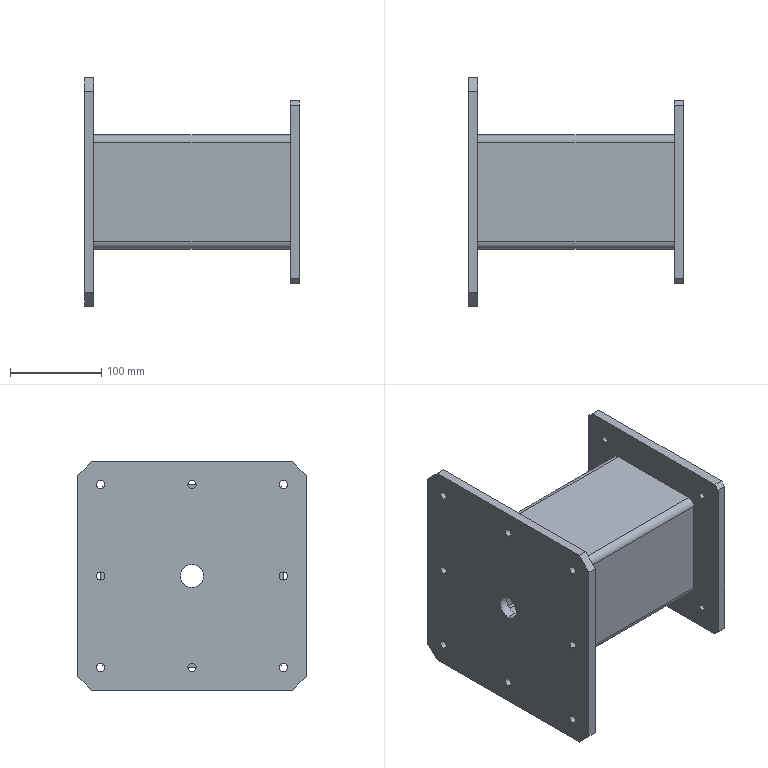Component | SolidWorks | Base-1 | 1 solid | 66 faces | box 235 x 250 x 250 mm | volume 1606520 mm3 | cylinder 36 | plane 30 | commonest cylinder face diameters 9 x16 7 x8 25 x4 16 x4 4 x4 | material Plain Carbon Steel
build123d program:
from build123d import *

# Parameters (mm, degrees)
SKETCH1_W                 = 400
SKETCH1_H                 = 400
BOSS_EXTRUDE1_DEPTH       = 20
BOSS_EXTRUDE2_DEPTH       = 430
SKETCH3_W                 = 500
SKETCH3_H                 = 500
BOSS_EXTRUDE3_DEPTH       = 20
CHAMFER1_SIZE             = 30
CHAMFER2_SIZE             = 10
M16_TAPPED_HOLE1_REACH    = 590.133
M16_TAPPED_HOLE1_BORE_R   = 7
M16_CLEARANCE_HOLE1_D     = 18
M16_CLEARANCE_HOLE1_DEPTH = 20
CUT_EXTRUDE1_DEPTH        = 589.133
CUT_EXTRUDE1_DEPTH_BACK   = 589.133
SKETCH11_R                = 25
SCALE1_SCALE              = 0.5


with BuildPart() as part:
    # Sketch1 → Boss-Extrude1 (new body)
    with BuildSketch(Plane.XY):
        Rectangle(SKETCH1_W, SKETCH1_H)
    extrude(amount=BOSS_EXTRUDE1_DEPTH)

    # Sketch2 → Boss-Extrude2 (add)
    with BuildSketch(Plane(origin=(0, 0, 0), x_dir=(-1, 0, 0), z_dir=(0, 0, -1))):
        with BuildLine():
            Line((-109, 125), (109, 125))
            ThreePointArc((109, 125), (120.314, 120.314), (125, 109))
            Line((125, 109), (125, -109))
            ThreePointArc((125, -109), (120.314, -120.314), (109, -125))
            Line((109, -125), (-109, -125))
            ThreePointArc((-109, -125), (-120.314, -120.314), (-125, -109))
            Line((-125, -109), (-125, 109))
            ThreePointArc((-125, 109), (-120.314, 120.314), (-109, 125))
        make_face()
        with BuildLine():
            Line((-109, 113), (109, 113))
            ThreePointArc((109, 113), (111.828, 111.828), (113, 109))
            Line((113, 109), (113, -109))
            ThreePointArc((113, -109), (111.828, -111.828), (109, -113))
            Line((109, -113), (-109, -113))
            ThreePointArc((-109, -113), (-111.828, -111.828), (-113, -109))
            Line((-113, -109), (-113, 109))
            ThreePointArc((-113, 109), (-111.828, 111.828), (-109, 113))
        make_face(mode=Mode.SUBTRACT)
    extrude(amount=BOSS_EXTRUDE2_DEPTH)

    # Sketch3 → Boss-Extrude3 (add)
    with BuildSketch(Plane(origin=(0, 0, -430), x_dir=(-1, 0, 0), z_dir=(0, 0, -1))):
        Rectangle(SKETCH3_W, SKETCH3_H)
    extrude(amount=BOSS_EXTRUDE3_DEPTH)

    # Chamfer1
    chamfer1_edges = [part.edges().sort_by_distance(p)[0] for p in [
        (-250, -250, -440),
        (-250, 250, -440),
        (250, 250, -440),
        (250, -250, -440),
    ]]
    chamfer(chamfer1_edges, length=CHAMFER1_SIZE)

    # Chamfer2
    chamfer2_edges = [part.edges().sort_by_distance(p)[0] for p in [
        (200, -200, 10),
        (-200, -200, 10),
        (-200, 200, 10),
        (200, 200, 10),
    ]]
    chamfer(chamfer2_edges, length=CHAMFER2_SIZE)

    # M16 Tapped Hole1 bore → M16 Tapped Hole1 (cut, up to next)
    with BuildSketch(Plane.XY.offset(20), mode=Mode.PRIVATE) as m16_tapped_hole1_sk1:
        with Locations((-150, -150)):
            Circle(M16_TAPPED_HOLE1_BORE_R)
    m16_tapped_hole1_tool1 = extrude(m16_tapped_hole1_sk1.sketch, amount=-M16_TAPPED_HOLE1_REACH, mode=Mode.PRIVATE) & part.part
    # M16 Tapped Hole1 bore → M16 Tapped Hole1 (cut, up to next)
    with BuildSketch(Plane.XY.offset(20), mode=Mode.PRIVATE) as m16_tapped_hole1_sk2:
        with Locations((-150, 150)):
            Circle(M16_TAPPED_HOLE1_BORE_R)
    m16_tapped_hole1_tool2 = extrude(m16_tapped_hole1_sk2.sketch, amount=-M16_TAPPED_HOLE1_REACH, mode=Mode.PRIVATE) & part.part
    # M16 Tapped Hole1 bore → M16 Tapped Hole1 (cut, up to next)
    with BuildSketch(Plane.XY.offset(20), mode=Mode.PRIVATE) as m16_tapped_hole1_sk3:
        with Locations((150, 150)):
            Circle(M16_TAPPED_HOLE1_BORE_R)
    m16_tapped_hole1_tool3 = extrude(m16_tapped_hole1_sk3.sketch, amount=-M16_TAPPED_HOLE1_REACH, mode=Mode.PRIVATE) & part.part
    # M16 Tapped Hole1 bore → M16 Tapped Hole1 (cut, up to next)
    with BuildSketch(Plane.XY.offset(20), mode=Mode.PRIVATE) as m16_tapped_hole1_sk4:
        with Locations((150, -150)):
            Circle(M16_TAPPED_HOLE1_BORE_R)
    m16_tapped_hole1_tool4 = extrude(m16_tapped_hole1_sk4.sketch, amount=-M16_TAPPED_HOLE1_REACH, mode=Mode.PRIVATE) & part.part
    add(m16_tapped_hole1_tool1.solids().sort_by_distance((-150, -150, 20))[0], mode=Mode.SUBTRACT)
    add(m16_tapped_hole1_tool2.solids().sort_by_distance((-150, 150, 20))[0], mode=Mode.SUBTRACT)
    add(m16_tapped_hole1_tool3.solids().sort_by_distance((150, 150, 20))[0], mode=Mode.SUBTRACT)
    add(m16_tapped_hole1_tool4.solids().sort_by_distance((150, -150, 20))[0], mode=Mode.SUBTRACT)

    # M16 Clearance Hole1
    with Locations(Plane.XY.offset(-430)):
        with Locations((-200, -200), (0, -200), (-200, 0), (0, 200), (-200, 200), (200, 200), (200, 0), (200, -200)):
            Hole(M16_CLEARANCE_HOLE1_D / 2, depth=M16_CLEARANCE_HOLE1_DEPTH)

    # Sketch11 → Cut-Extrude1 (cut, two sides: drawn at the far end of the back side and taken through both)
    with BuildSketch(Plane.XY.offset(20).offset(-CUT_EXTRUDE1_DEPTH_BACK)):
        Circle(SKETCH11_R)
    extrude(amount=CUT_EXTRUDE1_DEPTH + CUT_EXTRUDE1_DEPTH_BACK, mode=Mode.SUBTRACT)


with BuildPart() as part_1:
    # Scale1: scaled about (0, 0, 0)
    add(part.part.scale(SCALE1_SCALE))


solid = part_1.part

# Placed as in the assembly
solid = solid.moved(Location((-348.522, 19.945, 113.051), (0, 90, 0)))